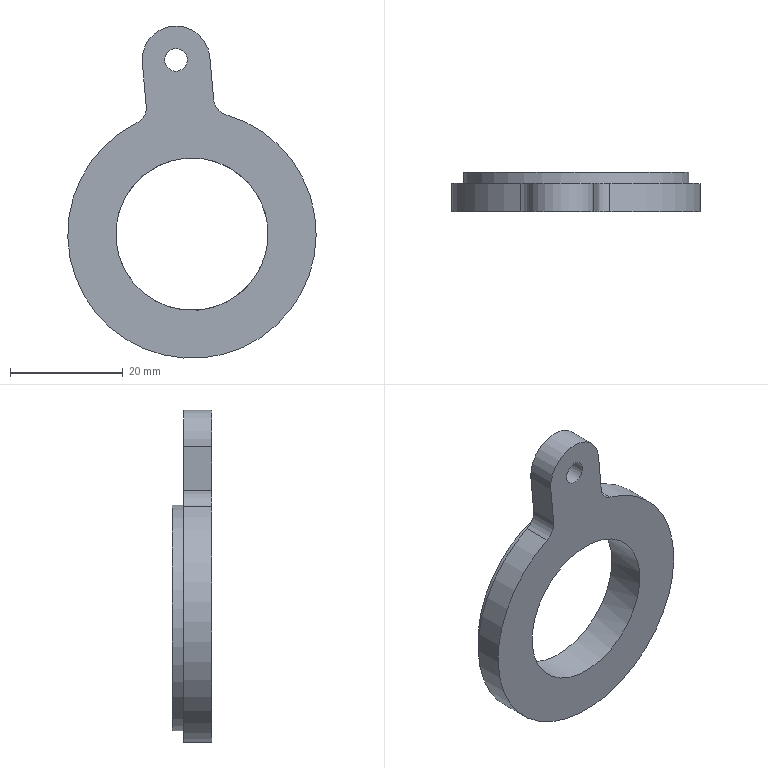Component | NX | SWIVEL_RING | 1 solid | 12 faces | volume 6893 mm3 | cylinder 7 | plane 5 | commonest cylinder face diameters 6 x2 44 x1 40 x1 27 x1 12 x1 4 x1